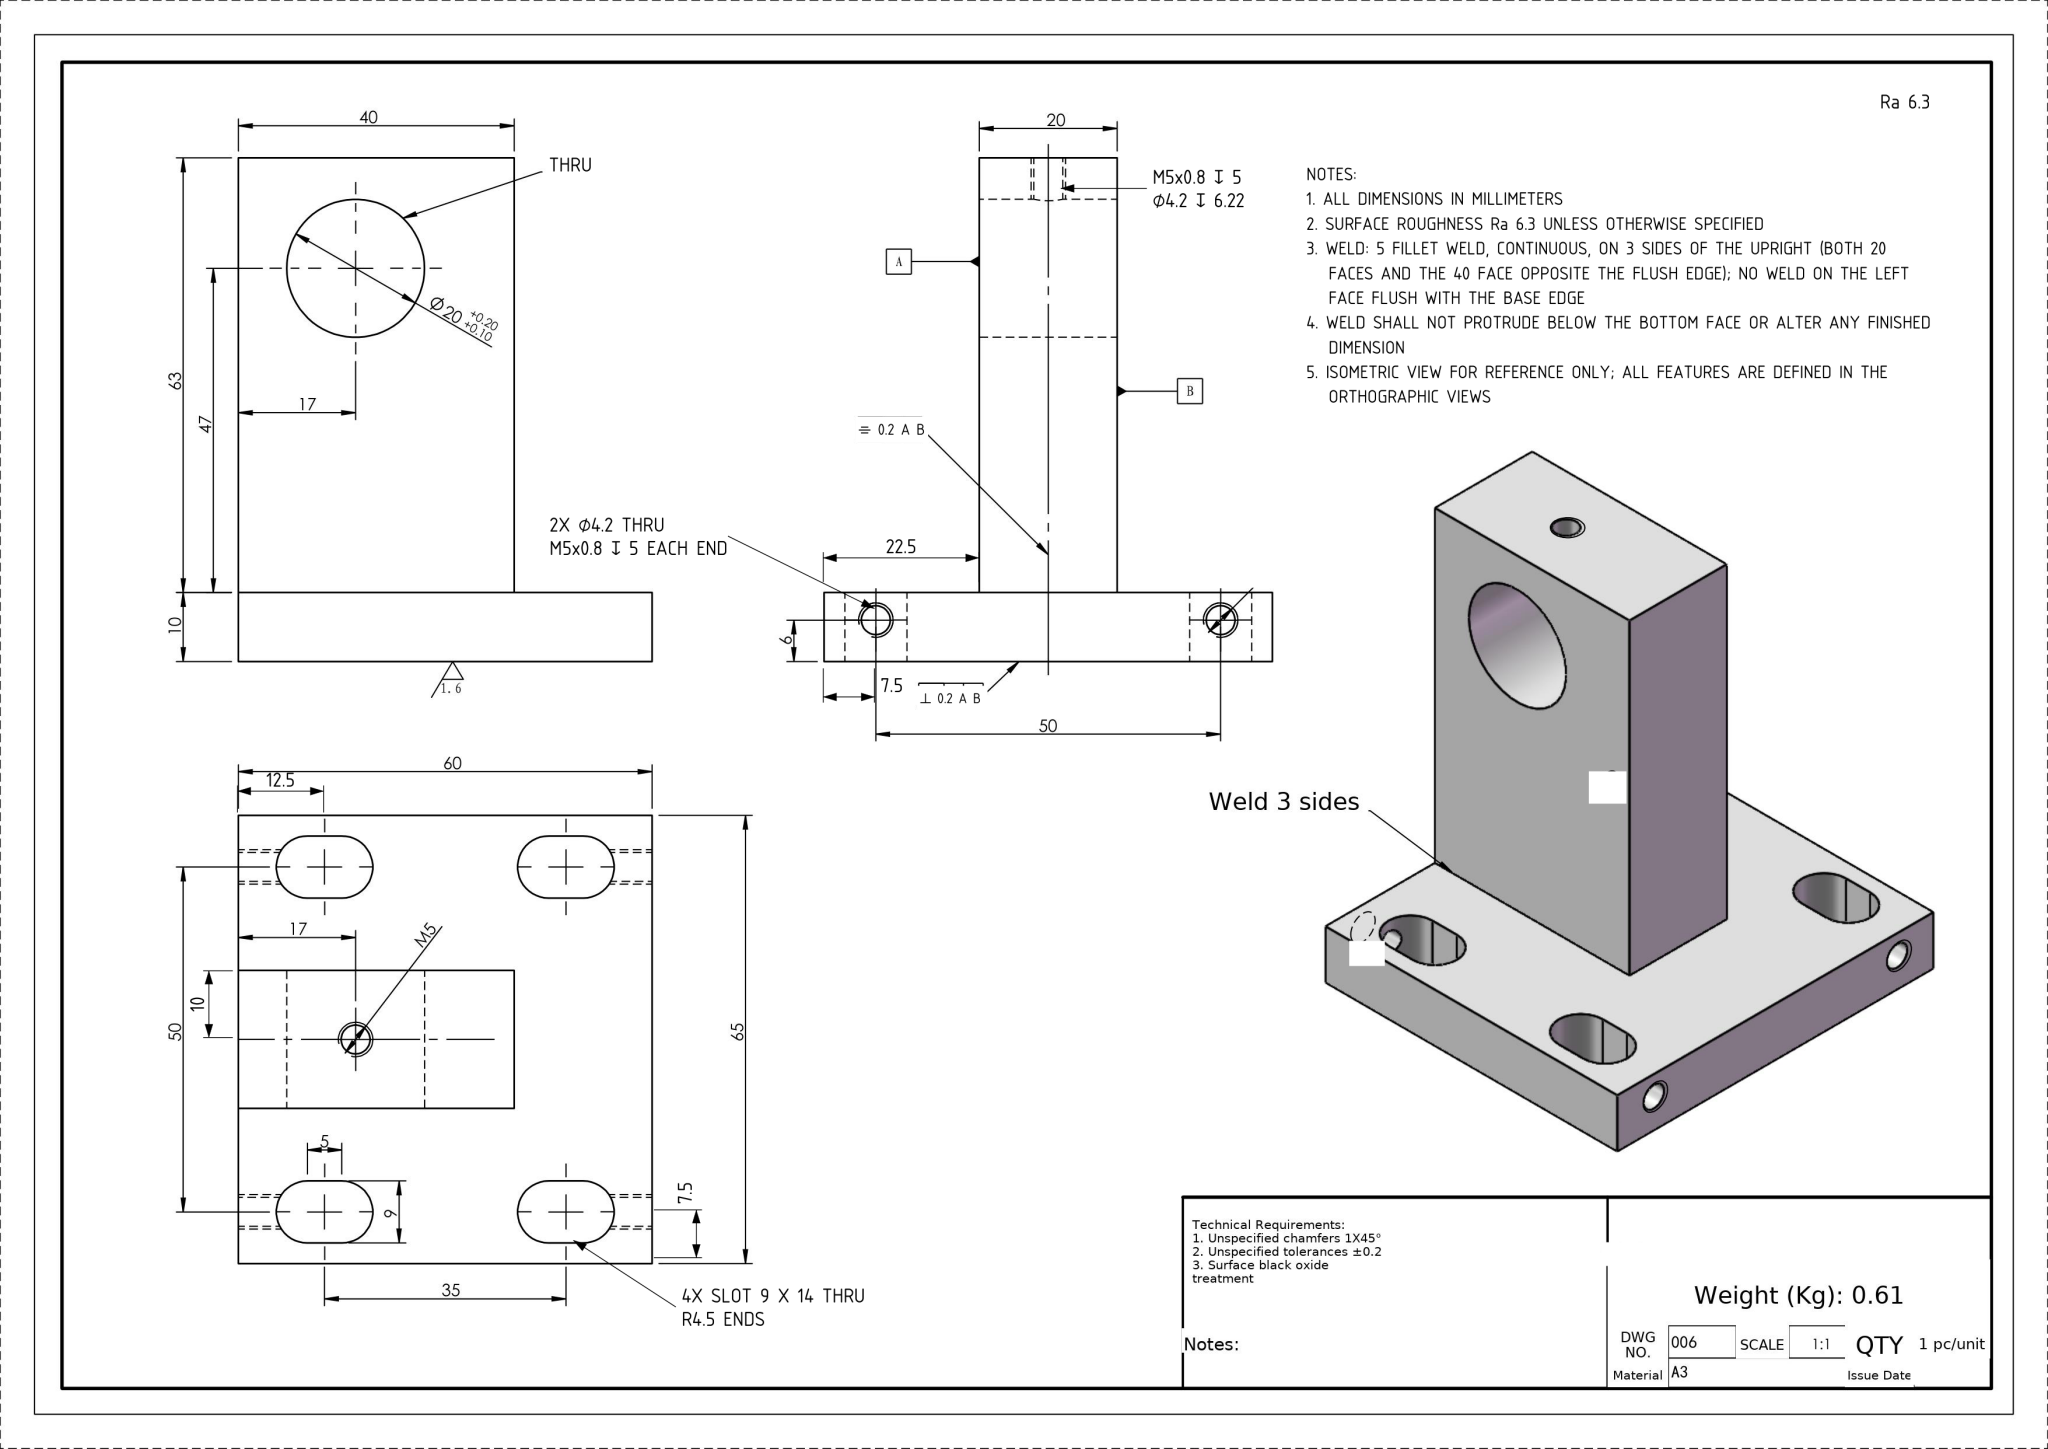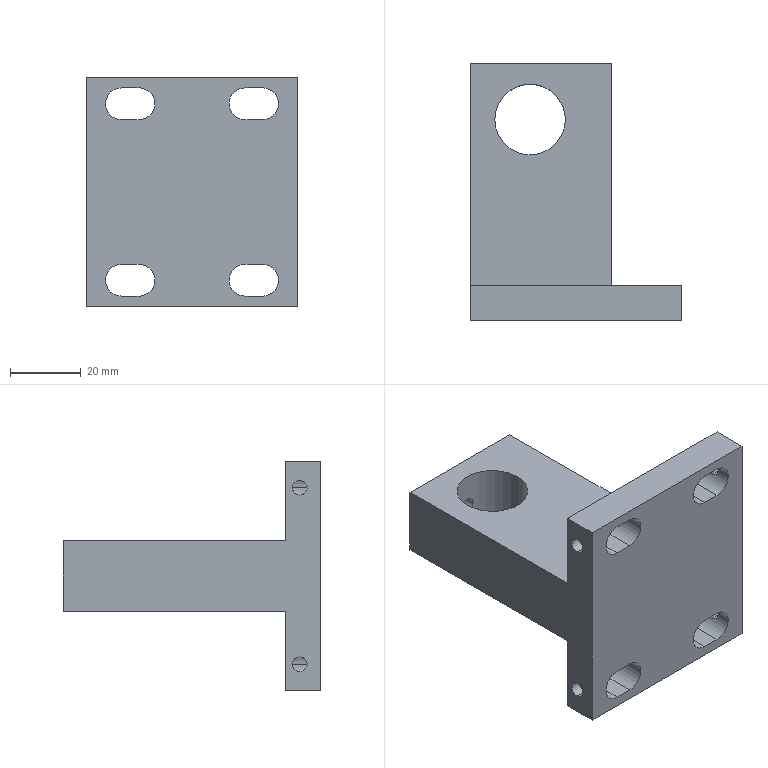Part | NX | mm | 1 solid | 42 faces | box 60 x 73 x 65 mm | volume 78377 mm3 | cylinder 24 | plane 18 | commonest cylinder face diameters 9 x12 4.2 x10 20 x2